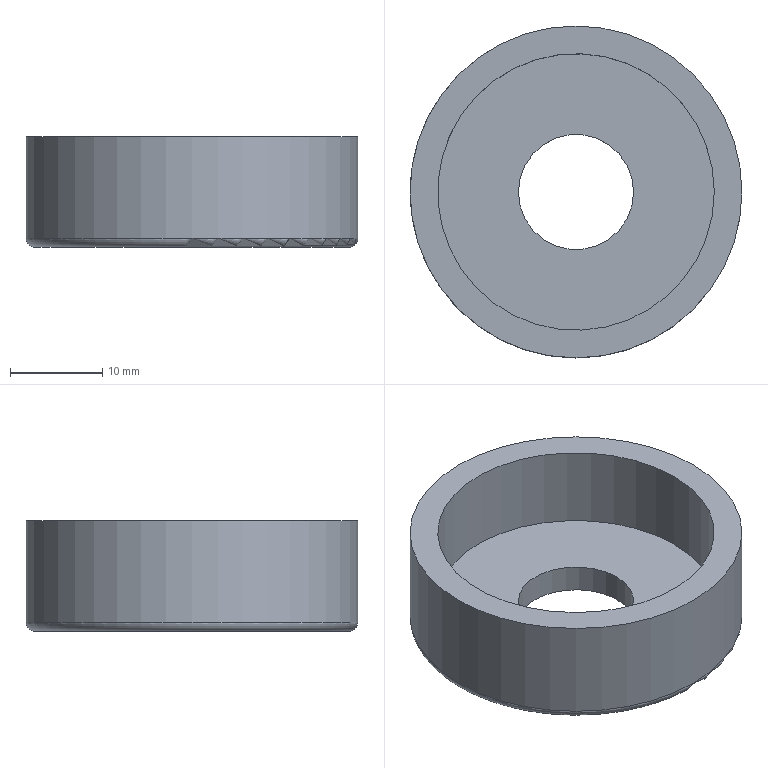Component | NX | SEATING_FOR_SPRING | 1 solid | 7 faces | box 36 x 36 x 12 mm | volume 5461 mm3 | cylinder 3 | plane 3 | torus 1 | commonest cylinder face diameters 36 x1 30 x1 12.5 x1
STEP:
#1=CARTESIAN_POINT('',(0.,0.,0.));
#2=DIRECTION('',(0.,0.,1.));
#3=DIRECTION('',(1.,0.,0.));
#4=AXIS2_PLACEMENT_3D('',#1,#2,#3);
#5=CARTESIAN_POINT('',(18.,0.,1.));
#6=VERTEX_POINT('',#5);
#7=CARTESIAN_POINT('',(0.,0.,1.));
#8=DIRECTION('',(0.,0.,1.));
#9=DIRECTION('',(1.,0.,0.));
#10=AXIS2_PLACEMENT_3D('',#7,#8,#9);
#11=CIRCLE('',#10,18.);
#12=CARTESIAN_POINT('',(0.,0.,12.));
#13=DIRECTION('',(0.,0.,-1.));
#14=DIRECTION('',(-1.,0.,0.));
#15=AXIS2_PLACEMENT_3D('',#12,#13,#14);
#16=CYLINDRICAL_SURFACE('',#15,18.);
#17=CARTESIAN_POINT('',(9.425,11.));
#18=DIRECTION('',(-1.,0.));
#19=VECTOR('',#18,1.);
#20=LINE('',#17,#19);
#21=(GEOMETRIC_REPRESENTATION_CONTEXT(2)PARAMETRIC_REPRESENTATION_CONTEXT()REPRESENTATION_CONTEXT('',''));
#22=DEFINITIONAL_REPRESENTATION('',(#20),#21);
#23=PCURVE('',#16,#22);
#24=CARTESIAN_POINT('',(0.,0.,1.));
#25=DIRECTION('',(0.,0.,1.));
#26=DIRECTION('',(1.,0.,0.));
#27=AXIS2_PLACEMENT_3D('',#24,#25,#26);
#28=TOROIDAL_SURFACE('',#27,17.,1.);
#29=CARTESIAN_POINT('',(0.,6.283));
#30=DIRECTION('',(1.,0.));
#31=VECTOR('',#30,1.);
#32=LINE('',#29,#31);
#33=(GEOMETRIC_REPRESENTATION_CONTEXT(2)PARAMETRIC_REPRESENTATION_CONTEXT()REPRESENTATION_CONTEXT('',''));
#34=DEFINITIONAL_REPRESENTATION('',(#32),#33);
#35=PCURVE('',#28,#34);
#36=SURFACE_CURVE('',#11,(#23,#35),.PCURVE_S1.);
#37=EDGE_CURVE('',#6,#6,#36,.T.);
#38=ORIENTED_EDGE('',*,*,#37,.T.);
#39=CARTESIAN_POINT('',(18.,0.,12.));
#40=VERTEX_POINT('',#39);
#41=CARTESIAN_POINT('',(18.,0.,12.));
#42=CARTESIAN_POINT('',(18.,0.,1.));
#43=B_SPLINE_CURVE_WITH_KNOTS('',1,(#41,#42),.UNSPECIFIED.,.F.,.F.,(2,2),(0.,11.),.PIECEWISE_BEZIER_KNOTS.);
#44=CARTESIAN_POINT('',(3.142,0.));
#45=DIRECTION('',(0.,1.));
#46=VECTOR('',#45,1.);
#47=LINE('',#44,#46);
#48=(GEOMETRIC_REPRESENTATION_CONTEXT(2)PARAMETRIC_REPRESENTATION_CONTEXT()REPRESENTATION_CONTEXT('',''));
#49=DEFINITIONAL_REPRESENTATION('',(#47),#48);
#50=PCURVE('',#16,#49);
#51=CARTESIAN_POINT('',(9.425,0.));
#52=DIRECTION('',(0.,1.));
#53=VECTOR('',#52,1.);
#54=LINE('',#51,#53);
#55=(GEOMETRIC_REPRESENTATION_CONTEXT(2)PARAMETRIC_REPRESENTATION_CONTEXT()REPRESENTATION_CONTEXT('',''));
#56=DEFINITIONAL_REPRESENTATION('',(#54),#55);
#57=PCURVE('',#16,#56);
#58=SEAM_CURVE('',#43,(#50,#57),.PCURVE_S1.);
#59=EDGE_CURVE('',#40,#6,#58,.T.);
#60=ORIENTED_EDGE('',*,*,#59,.F.);
#61=CARTESIAN_POINT('',(0.,0.,12.));
#62=DIRECTION('',(0.,0.,1.));
#63=DIRECTION('',(1.,0.,0.));
#64=AXIS2_PLACEMENT_3D('',#61,#62,#63);
#65=CIRCLE('',#64,18.);
#66=CARTESIAN_POINT('',(9.425,0.));
#67=DIRECTION('',(-1.,0.));
#68=VECTOR('',#67,1.);
#69=LINE('',#66,#68);
#70=(GEOMETRIC_REPRESENTATION_CONTEXT(2)PARAMETRIC_REPRESENTATION_CONTEXT()REPRESENTATION_CONTEXT('',''));
#71=DEFINITIONAL_REPRESENTATION('',(#69),#70);
#72=PCURVE('',#16,#71);
#73=CARTESIAN_POINT('',(0.,0.,12.));
#74=DIRECTION('',(0.,0.,1.));
#75=DIRECTION('',(1.,0.,0.));
#76=AXIS2_PLACEMENT_3D('',#73,#74,#75);
#77=PLANE('',#76);
#78=CARTESIAN_POINT('',(0.,0.));
#79=DIRECTION('',(1.,0.));
#80=AXIS2_PLACEMENT_2D('',#78,#79);
#81=CIRCLE('',#80,18.);
#82=(GEOMETRIC_REPRESENTATION_CONTEXT(2)PARAMETRIC_REPRESENTATION_CONTEXT()REPRESENTATION_CONTEXT('',''));
#83=DEFINITIONAL_REPRESENTATION('',(#81),#82);
#84=PCURVE('',#77,#83);
#85=SURFACE_CURVE('',#65,(#72,#84),.PCURVE_S1.);
#86=EDGE_CURVE('',#40,#40,#85,.T.);
#87=ORIENTED_EDGE('',*,*,#86,.F.);
#88=ORIENTED_EDGE('',*,*,#59,.T.);
#89=EDGE_LOOP('',(#38,#60,#87,#88));
#90=FACE_BOUND('',#89,.T.);
#91=ADVANCED_FACE('',(#90),#16,.T.);
#92=CARTESIAN_POINT('',(15.,0.,12.));
#93=VERTEX_POINT('',#92);
#94=CARTESIAN_POINT('',(0.,0.,12.));
#95=DIRECTION('',(0.,0.,1.));
#96=DIRECTION('',(1.,0.,0.));
#97=AXIS2_PLACEMENT_3D('',#94,#95,#96);
#98=CIRCLE('',#97,15.);
#99=CARTESIAN_POINT('',(0.,0.));
#100=DIRECTION('',(1.,0.));
#101=AXIS2_PLACEMENT_2D('',#99,#100);
#102=CIRCLE('',#101,15.);
#103=(GEOMETRIC_REPRESENTATION_CONTEXT(2)PARAMETRIC_REPRESENTATION_CONTEXT()REPRESENTATION_CONTEXT('',''));
#104=DEFINITIONAL_REPRESENTATION('',(#102),#103);
#105=PCURVE('',#77,#104);
#106=CARTESIAN_POINT('',(0.,0.,12.));
#107=DIRECTION('',(0.,0.,-1.));
#108=DIRECTION('',(-1.,0.,0.));
#109=AXIS2_PLACEMENT_3D('',#106,#107,#108);
#110=CYLINDRICAL_SURFACE('',#109,15.);
#111=CARTESIAN_POINT('',(9.425,0.));
#112=DIRECTION('',(-1.,0.));
#113=VECTOR('',#112,1.);
#114=LINE('',#111,#113);
#115=(GEOMETRIC_REPRESENTATION_CONTEXT(2)PARAMETRIC_REPRESENTATION_CONTEXT()REPRESENTATION_CONTEXT('',''));
#116=DEFINITIONAL_REPRESENTATION('',(#114),#115);
#117=PCURVE('',#110,#116);
#118=SURFACE_CURVE('',#98,(#105,#117),.PCURVE_S1.);
#119=EDGE_CURVE('',#93,#93,#118,.T.);
#120=ORIENTED_EDGE('',*,*,#119,.F.);
#121=EDGE_LOOP('',(#120));
#122=FACE_BOUND('',#121,.T.);
#123=ORIENTED_EDGE('',*,*,#86,.T.);
#124=EDGE_LOOP('',(#123));
#125=FACE_BOUND('',#124,.T.);
#126=ADVANCED_FACE('',(#122,#125),#77,.T.);
#127=CARTESIAN_POINT('',(17.,0.,0.));
#128=VERTEX_POINT('',#127);
#129=CARTESIAN_POINT('',(0.,0.,0.));
#130=DIRECTION('',(0.,0.,-1.));
#131=DIRECTION('',(1.,0.,0.));
#132=AXIS2_PLACEMENT_3D('',#129,#130,#131);
#133=CIRCLE('',#132,17.);
#134=CARTESIAN_POINT('',(0.,0.,0.));
#135=DIRECTION('',(0.,0.,1.));
#136=DIRECTION('',(1.,0.,0.));
#137=AXIS2_PLACEMENT_3D('',#134,#135,#136);
#138=PLANE('',#137);
#139=CARTESIAN_POINT('',(17.,0.));
#140=CARTESIAN_POINT('',(17.,-29.445));
#141=CARTESIAN_POINT('',(-8.5,-14.722));
#142=CARTESIAN_POINT('',(-34.,-0.));
#143=CARTESIAN_POINT('',(-8.5,14.722));
#144=CARTESIAN_POINT('',(17.,29.445));
#145=CARTESIAN_POINT('',(17.,0.));
#146=(BOUNDED_CURVE()B_SPLINE_CURVE(2,(#139,#140,#141,#142,#143,#144,#145),.UNSPECIFIED.,.T.,.F.)B_SPLINE_CURVE_WITH_KNOTS((1,2,2,2,2,1),(-2.094,0.,2.094,4.189,6.283,8.378),.UNSPECIFIED.)CURVE()GEOMETRIC_REPRESENTATION_ITEM()RATIONAL_B_SPLINE_CURVE((1.,0.5,1.,0.5,1.,0.5,1.))REPRESENTATION_ITEM(''));
#147=(GEOMETRIC_REPRESENTATION_CONTEXT(2)PARAMETRIC_REPRESENTATION_CONTEXT()REPRESENTATION_CONTEXT('',''));
#148=DEFINITIONAL_REPRESENTATION('',(#146),#147);
#149=PCURVE('',#138,#148);
#150=CARTESIAN_POINT('',(6.283,4.712));
#151=DIRECTION('',(-1.,0.));
#152=VECTOR('',#151,1.);
#153=LINE('',#150,#152);
#154=(GEOMETRIC_REPRESENTATION_CONTEXT(2)PARAMETRIC_REPRESENTATION_CONTEXT()REPRESENTATION_CONTEXT('',''));
#155=DEFINITIONAL_REPRESENTATION('',(#153),#154);
#156=PCURVE('',#28,#155);
#157=SURFACE_CURVE('',#133,(#149,#156),.PCURVE_S1.);
#158=EDGE_CURVE('',#128,#128,#157,.T.);
#159=ORIENTED_EDGE('',*,*,#158,.T.);
#160=EDGE_LOOP('',(#159));
#161=FACE_BOUND('',#160,.T.);
#162=CARTESIAN_POINT('',(-6.25,0.,0.));
#163=VERTEX_POINT('',#162);
#164=CARTESIAN_POINT('',(0.,0.,0.));
#165=DIRECTION('',(0.,0.,-1.));
#166=DIRECTION('',(-1.,0.,0.));
#167=AXIS2_PLACEMENT_3D('',#164,#165,#166);
#168=CIRCLE('',#167,6.25);
#169=CARTESIAN_POINT('',(-6.25,0.));
#170=CARTESIAN_POINT('',(-6.25,10.825));
#171=CARTESIAN_POINT('',(3.125,5.413));
#172=CARTESIAN_POINT('',(12.5,0.));
#173=CARTESIAN_POINT('',(3.125,-5.413));
#174=CARTESIAN_POINT('',(-6.25,-10.825));
#175=CARTESIAN_POINT('',(-6.25,0.));
#176=(BOUNDED_CURVE()B_SPLINE_CURVE(2,(#169,#170,#171,#172,#173,#174,#175),.UNSPECIFIED.,.T.,.F.)B_SPLINE_CURVE_WITH_KNOTS((1,2,2,2,2,1),(-2.094,0.,2.094,4.189,6.283,8.378),.UNSPECIFIED.)CURVE()GEOMETRIC_REPRESENTATION_ITEM()RATIONAL_B_SPLINE_CURVE((1.,0.5,1.,0.5,1.,0.5,1.))REPRESENTATION_ITEM(''));
#177=(GEOMETRIC_REPRESENTATION_CONTEXT(2)PARAMETRIC_REPRESENTATION_CONTEXT()REPRESENTATION_CONTEXT('',''));
#178=DEFINITIONAL_REPRESENTATION('',(#176),#177);
#179=PCURVE('',#138,#178);
#180=CARTESIAN_POINT('',(0.,0.,3.));
#181=DIRECTION('',(0.,0.,-1.));
#182=DIRECTION('',(-1.,0.,0.));
#183=AXIS2_PLACEMENT_3D('',#180,#181,#182);
#184=CYLINDRICAL_SURFACE('',#183,6.25);
#185=CARTESIAN_POINT('',(0.,3.));
#186=DIRECTION('',(1.,0.));
#187=VECTOR('',#186,1.);
#188=LINE('',#185,#187);
#189=(GEOMETRIC_REPRESENTATION_CONTEXT(2)PARAMETRIC_REPRESENTATION_CONTEXT()REPRESENTATION_CONTEXT('',''));
#190=DEFINITIONAL_REPRESENTATION('',(#188),#189);
#191=PCURVE('',#184,#190);
#192=SURFACE_CURVE('',#168,(#179,#191),.PCURVE_S1.);
#193=EDGE_CURVE('',#163,#163,#192,.T.);
#194=ORIENTED_EDGE('',*,*,#193,.F.);
#195=EDGE_LOOP('',(#194));
#196=FACE_BOUND('',#195,.T.);
#197=ADVANCED_FACE('',(#161,#196),#138,.F.);
#198=ORIENTED_EDGE('',*,*,#119,.F.);
#199=CARTESIAN_POINT('',(15.,0.,3.));
#200=VERTEX_POINT('',#199);
#201=CARTESIAN_POINT('',(15.,0.,12.));
#202=CARTESIAN_POINT('',(15.,0.,3.));
#203=B_SPLINE_CURVE_WITH_KNOTS('',1,(#201,#202),.UNSPECIFIED.,.F.,.F.,(2,2),(0.,9.),.PIECEWISE_BEZIER_KNOTS.);
#204=CARTESIAN_POINT('',(9.425,0.));
#205=DIRECTION('',(0.,1.));
#206=VECTOR('',#205,1.);
#207=LINE('',#204,#206);
#208=(GEOMETRIC_REPRESENTATION_CONTEXT(2)PARAMETRIC_REPRESENTATION_CONTEXT()REPRESENTATION_CONTEXT('',''));
#209=DEFINITIONAL_REPRESENTATION('',(#207),#208);
#210=PCURVE('',#110,#209);
#211=CARTESIAN_POINT('',(3.142,0.));
#212=DIRECTION('',(0.,1.));
#213=VECTOR('',#212,1.);
#214=LINE('',#211,#213);
#215=(GEOMETRIC_REPRESENTATION_CONTEXT(2)PARAMETRIC_REPRESENTATION_CONTEXT()REPRESENTATION_CONTEXT('',''));
#216=DEFINITIONAL_REPRESENTATION('',(#214),#215);
#217=PCURVE('',#110,#216);
#218=SEAM_CURVE('',#203,(#210,#217),.PCURVE_S1.);
#219=EDGE_CURVE('',#93,#200,#218,.T.);
#220=ORIENTED_EDGE('',*,*,#219,.T.);
#221=CARTESIAN_POINT('',(0.,0.,3.));
#222=DIRECTION('',(0.,0.,1.));
#223=DIRECTION('',(1.,0.,0.));
#224=AXIS2_PLACEMENT_3D('',#221,#222,#223);
#225=CIRCLE('',#224,15.);
#226=CARTESIAN_POINT('',(9.425,9.));
#227=DIRECTION('',(-1.,0.));
#228=VECTOR('',#227,1.);
#229=LINE('',#226,#228);
#230=(GEOMETRIC_REPRESENTATION_CONTEXT(2)PARAMETRIC_REPRESENTATION_CONTEXT()REPRESENTATION_CONTEXT('',''));
#231=DEFINITIONAL_REPRESENTATION('',(#229),#230);
#232=PCURVE('',#110,#231);
#233=CARTESIAN_POINT('',(0.,0.,3.));
#234=DIRECTION('',(0.,0.,1.));
#235=DIRECTION('',(1.,0.,0.));
#236=AXIS2_PLACEMENT_3D('',#233,#234,#235);
#237=PLANE('',#236);
#238=CARTESIAN_POINT('',(0.,0.));
#239=DIRECTION('',(1.,0.));
#240=AXIS2_PLACEMENT_2D('',#238,#239);
#241=CIRCLE('',#240,15.);
#242=(GEOMETRIC_REPRESENTATION_CONTEXT(2)PARAMETRIC_REPRESENTATION_CONTEXT()REPRESENTATION_CONTEXT('',''));
#243=DEFINITIONAL_REPRESENTATION('',(#241),#242);
#244=PCURVE('',#237,#243);
#245=SURFACE_CURVE('',#225,(#232,#244),.PCURVE_S1.);
#246=EDGE_CURVE('',#200,#200,#245,.T.);
#247=ORIENTED_EDGE('',*,*,#246,.T.);
#248=ORIENTED_EDGE('',*,*,#219,.F.);
#249=EDGE_LOOP('',(#198,#220,#247,#248));
#250=FACE_BOUND('',#249,.F.);
#251=ADVANCED_FACE('',(#250),#110,.F.);
#252=CARTESIAN_POINT('',(-6.25,0.,3.));
#253=VERTEX_POINT('',#252);
#254=CARTESIAN_POINT('',(0.,0.,3.));
#255=DIRECTION('',(0.,0.,-1.));
#256=DIRECTION('',(-1.,0.,0.));
#257=AXIS2_PLACEMENT_3D('',#254,#255,#256);
#258=CIRCLE('',#257,6.25);
#259=CARTESIAN_POINT('',(-6.25,0.));
#260=CARTESIAN_POINT('',(-6.25,10.825));
#261=CARTESIAN_POINT('',(3.125,5.413));
#262=CARTESIAN_POINT('',(12.5,0.));
#263=CARTESIAN_POINT('',(3.125,-5.413));
#264=CARTESIAN_POINT('',(-6.25,-10.825));
#265=CARTESIAN_POINT('',(-6.25,0.));
#266=(BOUNDED_CURVE()B_SPLINE_CURVE(2,(#259,#260,#261,#262,#263,#264,#265),.UNSPECIFIED.,.T.,.F.)B_SPLINE_CURVE_WITH_KNOTS((1,2,2,2,2,1),(-2.094,0.,2.094,4.189,6.283,8.378),.UNSPECIFIED.)CURVE()GEOMETRIC_REPRESENTATION_ITEM()RATIONAL_B_SPLINE_CURVE((1.,0.5,1.,0.5,1.,0.5,1.))REPRESENTATION_ITEM(''));
#267=(GEOMETRIC_REPRESENTATION_CONTEXT(2)PARAMETRIC_REPRESENTATION_CONTEXT()REPRESENTATION_CONTEXT('',''));
#268=DEFINITIONAL_REPRESENTATION('',(#266),#267);
#269=PCURVE('',#237,#268);
#270=CARTESIAN_POINT('',(0.,0.));
#271=DIRECTION('',(1.,0.));
#272=VECTOR('',#271,1.);
#273=LINE('',#270,#272);
#274=(GEOMETRIC_REPRESENTATION_CONTEXT(2)PARAMETRIC_REPRESENTATION_CONTEXT()REPRESENTATION_CONTEXT('',''));
#275=DEFINITIONAL_REPRESENTATION('',(#273),#274);
#276=PCURVE('',#184,#275);
#277=SURFACE_CURVE('',#258,(#269,#276),.PCURVE_S1.);
#278=EDGE_CURVE('',#253,#253,#277,.T.);
#279=ORIENTED_EDGE('',*,*,#278,.T.);
#280=EDGE_LOOP('',(#279));
#281=FACE_BOUND('',#280,.T.);
#282=ORIENTED_EDGE('',*,*,#246,.T.);
#283=EDGE_LOOP('',(#282));
#284=FACE_BOUND('',#283,.T.);
#285=ADVANCED_FACE('',(#281,#284),#237,.T.);
#286=ORIENTED_EDGE('',*,*,#193,.F.);
#287=CARTESIAN_POINT('',(-6.25,-0.,3.));
#288=CARTESIAN_POINT('',(-6.25,-0.,0.));
#289=B_SPLINE_CURVE_WITH_KNOTS('',1,(#287,#288),.UNSPECIFIED.,.F.,.F.,(2,2),(0.,3.),.PIECEWISE_BEZIER_KNOTS.);
#290=CARTESIAN_POINT('',(0.,0.));
#291=DIRECTION('',(0.,1.));
#292=VECTOR('',#291,1.);
#293=LINE('',#290,#292);
#294=(GEOMETRIC_REPRESENTATION_CONTEXT(2)PARAMETRIC_REPRESENTATION_CONTEXT()REPRESENTATION_CONTEXT('',''));
#295=DEFINITIONAL_REPRESENTATION('',(#293),#294);
#296=PCURVE('',#184,#295);
#297=CARTESIAN_POINT('',(6.283,0.));
#298=DIRECTION('',(0.,1.));
#299=VECTOR('',#298,1.);
#300=LINE('',#297,#299);
#301=(GEOMETRIC_REPRESENTATION_CONTEXT(2)PARAMETRIC_REPRESENTATION_CONTEXT()REPRESENTATION_CONTEXT('',''));
#302=DEFINITIONAL_REPRESENTATION('',(#300),#301);
#303=PCURVE('',#184,#302);
#304=SEAM_CURVE('',#289,(#296,#303),.PCURVE_S1.);
#305=EDGE_CURVE('',#253,#163,#304,.T.);
#306=ORIENTED_EDGE('',*,*,#305,.F.);
#307=ORIENTED_EDGE('',*,*,#278,.T.);
#308=ORIENTED_EDGE('',*,*,#305,.T.);
#309=EDGE_LOOP('',(#286,#306,#307,#308));
#310=FACE_BOUND('',#309,.F.);
#311=ADVANCED_FACE('',(#310),#184,.F.);
#312=ORIENTED_EDGE('',*,*,#158,.F.);
#313=CARTESIAN_POINT('',(17.,0.,0.));
#314=CARTESIAN_POINT('',(17.267,0.,0.));
#315=CARTESIAN_POINT('',(17.528,0.,0.085));
#316=CARTESIAN_POINT('',(17.752,0.,0.2481));
#317=CARTESIAN_POINT('',(17.915,0.,0.4723));
#318=CARTESIAN_POINT('',(18.,0.,0.7327));
#319=CARTESIAN_POINT('',(18.,0.,1.));
#320=(BOUNDED_CURVE()B_SPLINE_CURVE(6,(#313,#314,#315,#316,#317,#318,#319),.UNSPECIFIED.,.F.,.F.)B_SPLINE_CURVE_WITH_KNOTS((7,7),(4.712,6.283),.PIECEWISE_BEZIER_KNOTS.)CURVE()GEOMETRIC_REPRESENTATION_ITEM()RATIONAL_B_SPLINE_CURVE((1.031,1.01,0.9979,0.994,0.9979,1.01,1.031))REPRESENTATION_ITEM(''));
#321=CARTESIAN_POINT('',(6.283,0.));
#322=DIRECTION('',(0.,1.));
#323=VECTOR('',#322,1.);
#324=LINE('',#321,#323);
#325=(GEOMETRIC_REPRESENTATION_CONTEXT(2)PARAMETRIC_REPRESENTATION_CONTEXT()REPRESENTATION_CONTEXT('',''));
#326=DEFINITIONAL_REPRESENTATION('',(#324),#325);
#327=PCURVE('',#28,#326);
#328=CARTESIAN_POINT('',(0.,0.));
#329=DIRECTION('',(0.,1.));
#330=VECTOR('',#329,1.);
#331=LINE('',#328,#330);
#332=(GEOMETRIC_REPRESENTATION_CONTEXT(2)PARAMETRIC_REPRESENTATION_CONTEXT()REPRESENTATION_CONTEXT('',''));
#333=DEFINITIONAL_REPRESENTATION('',(#331),#332);
#334=PCURVE('',#28,#333);
#335=SEAM_CURVE('',#320,(#327,#334),.PCURVE_S1.);
#336=EDGE_CURVE('',#128,#6,#335,.T.);
#337=ORIENTED_EDGE('',*,*,#336,.T.);
#338=ORIENTED_EDGE('',*,*,#37,.F.);
#339=ORIENTED_EDGE('',*,*,#336,.F.);
#340=EDGE_LOOP('',(#312,#337,#338,#339));
#341=FACE_BOUND('',#340,.T.);
#342=ADVANCED_FACE('',(#341),#28,.T.);
#343=CLOSED_SHELL('',(#91,#126,#197,#251,#285,#311,#342));
#344=MANIFOLD_SOLID_BREP('',#343);
#345=(LENGTH_UNIT()NAMED_UNIT(*)SI_UNIT(.MILLI.,.METRE.));
#346=UNCERTAINTY_MEASURE_WITH_UNIT(LENGTH_MEASURE(0.00001),#345,'','');
#347=(NAMED_UNIT(*)PLANE_ANGLE_UNIT()SI_UNIT($,.RADIAN.));
#348=(NAMED_UNIT(*)SI_UNIT($,.STERADIAN.)SOLID_ANGLE_UNIT());
#349=(GEOMETRIC_REPRESENTATION_CONTEXT(3)GLOBAL_UNCERTAINTY_ASSIGNED_CONTEXT((#346))GLOBAL_UNIT_ASSIGNED_CONTEXT((#345,#347,#348))REPRESENTATION_CONTEXT('',''));
#350=ADVANCED_BREP_SHAPE_REPRESENTATION('',(#4,#344),#349);